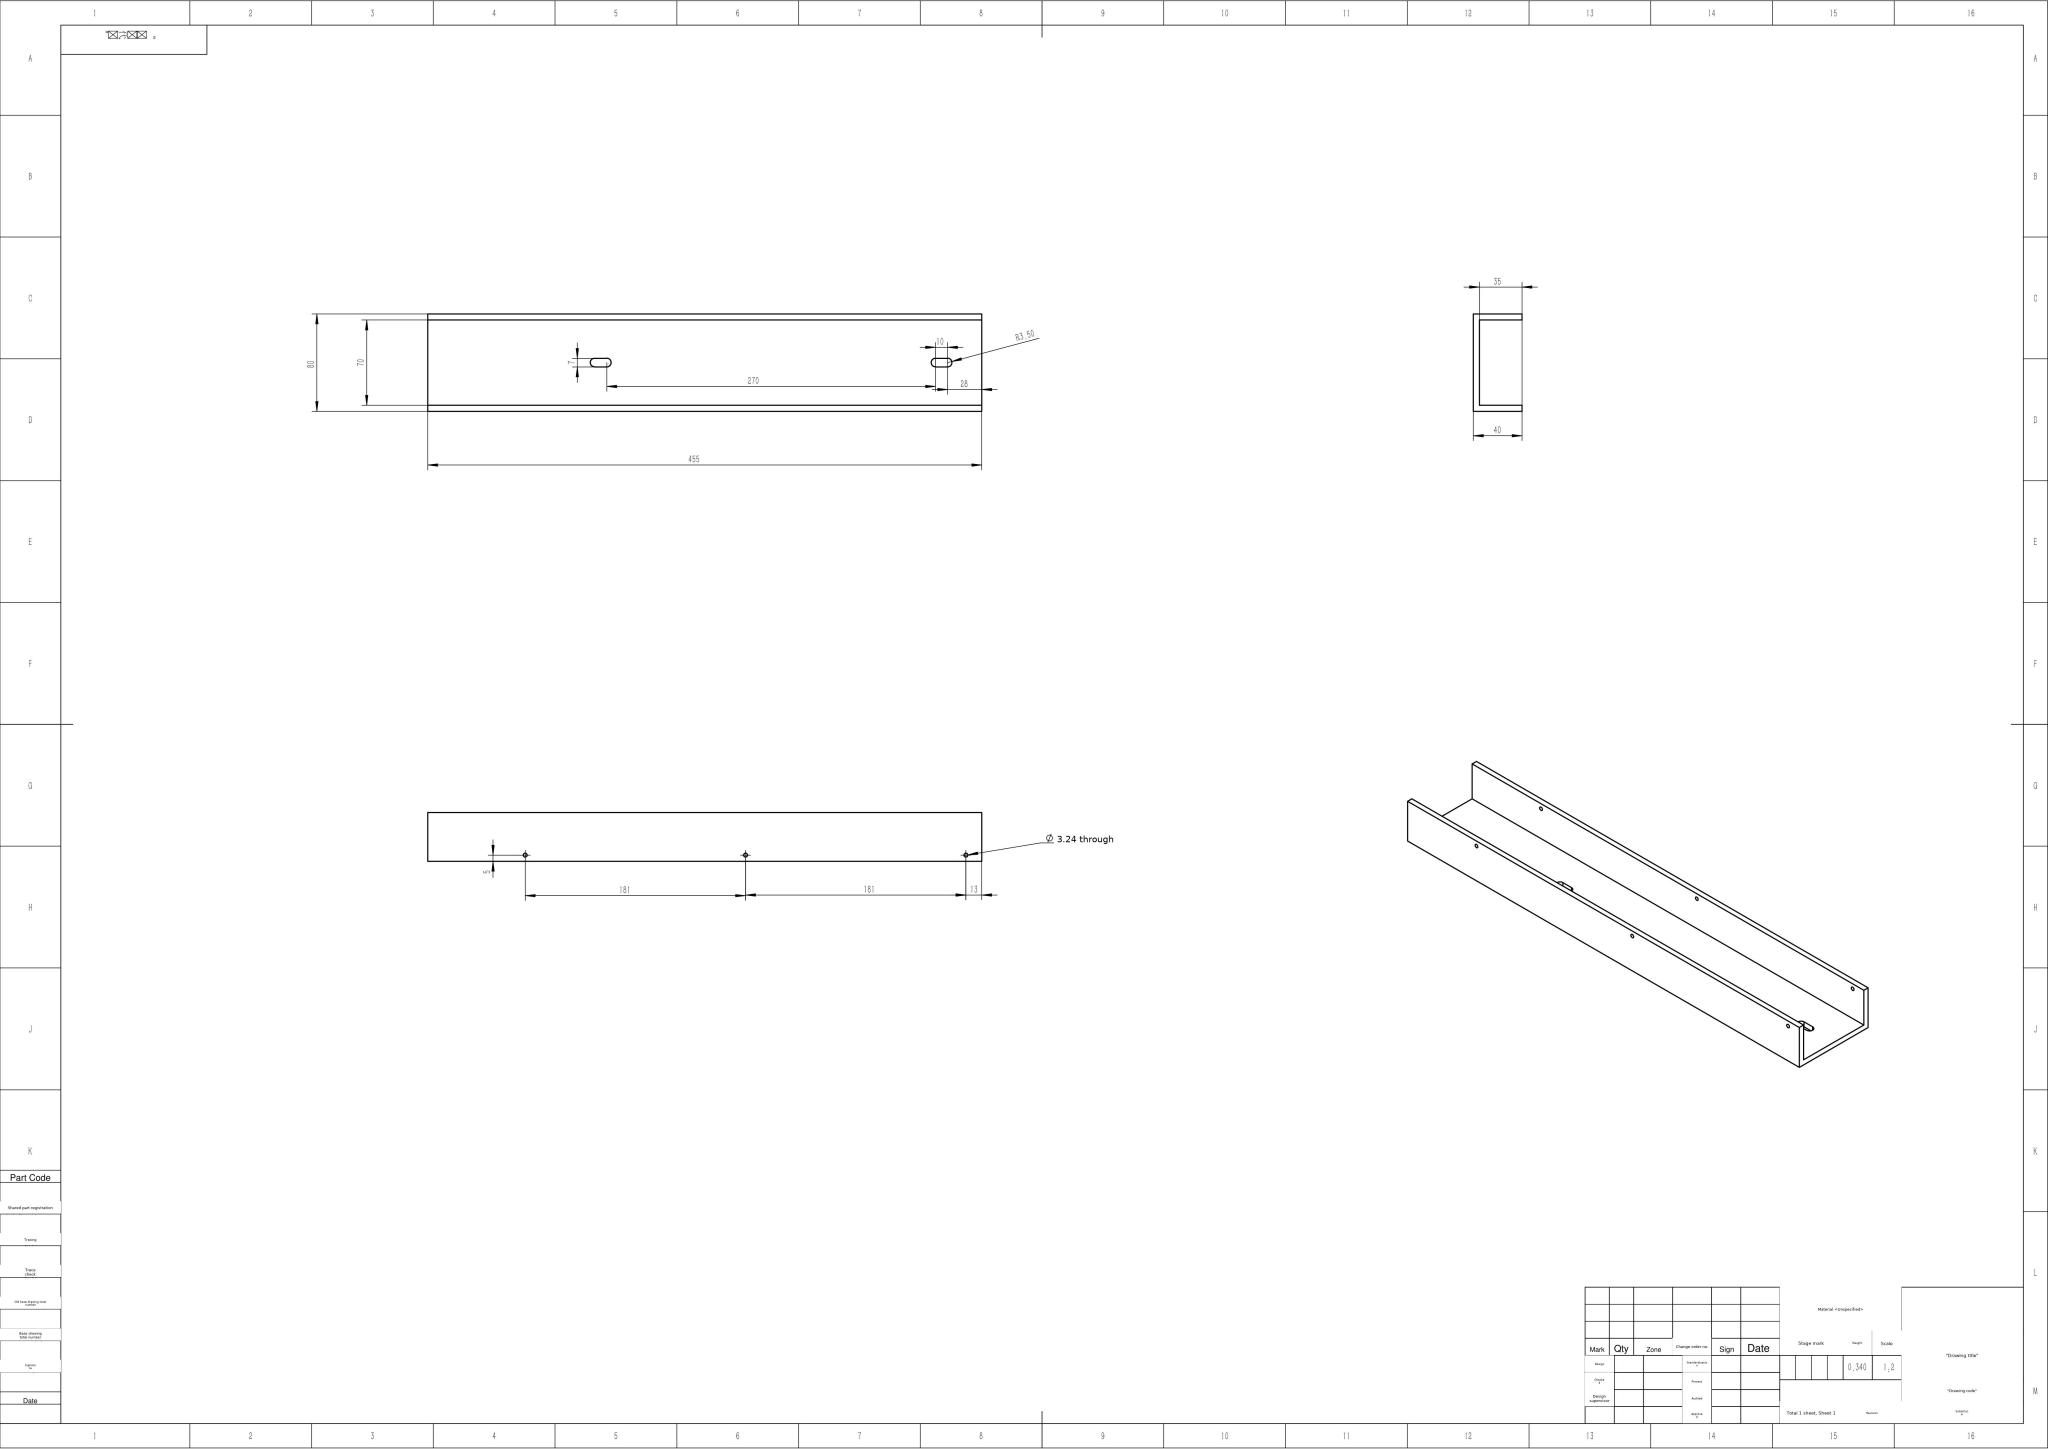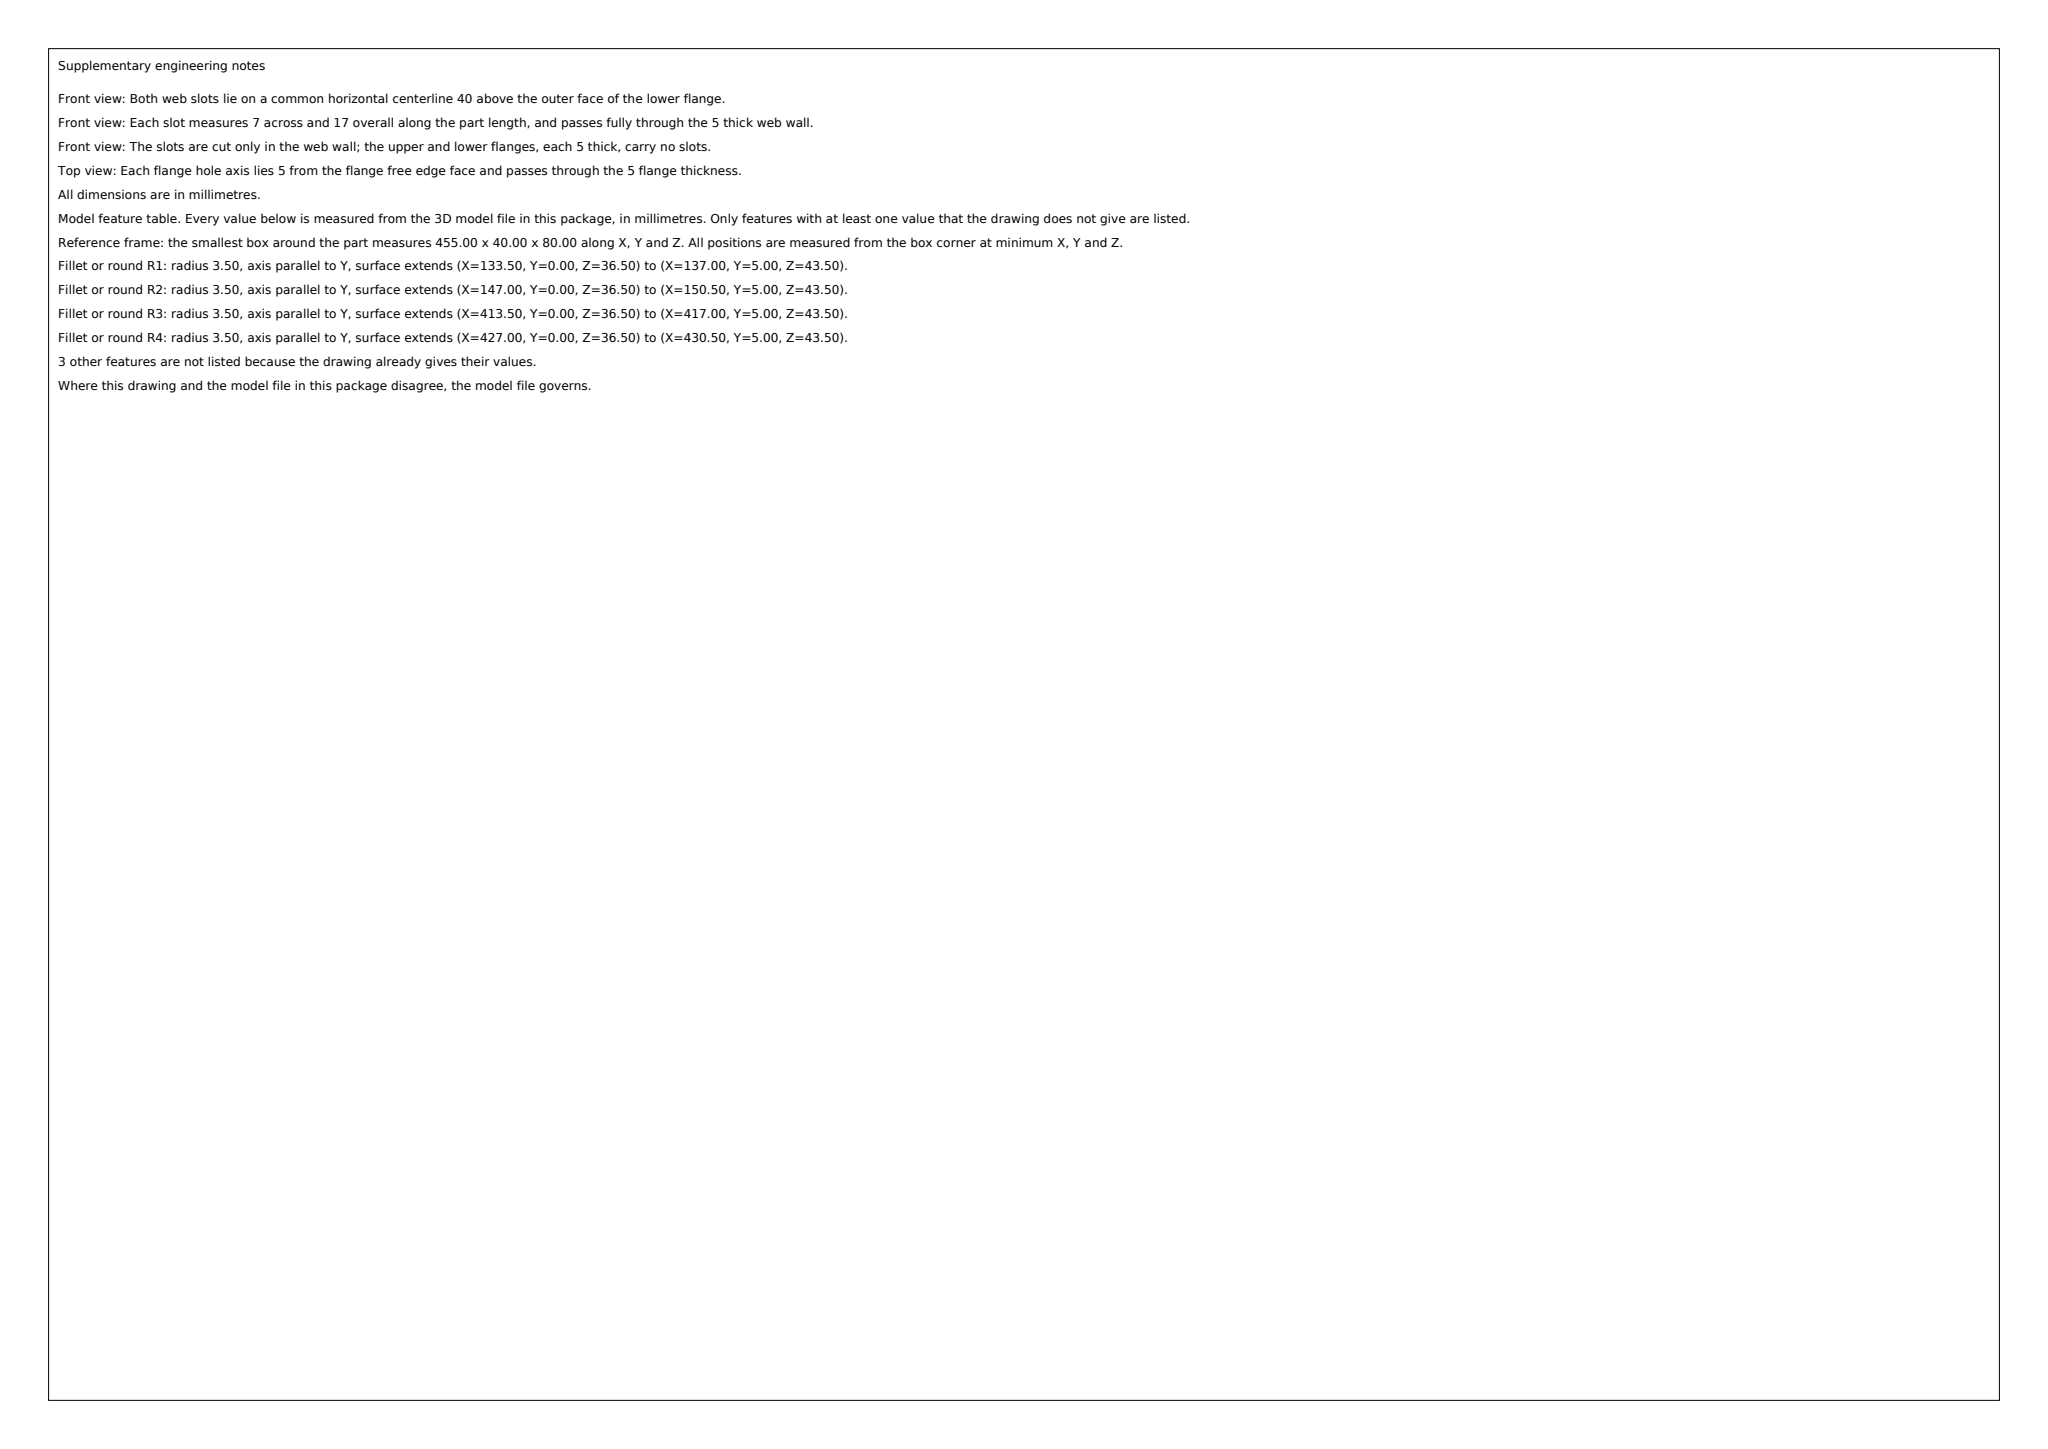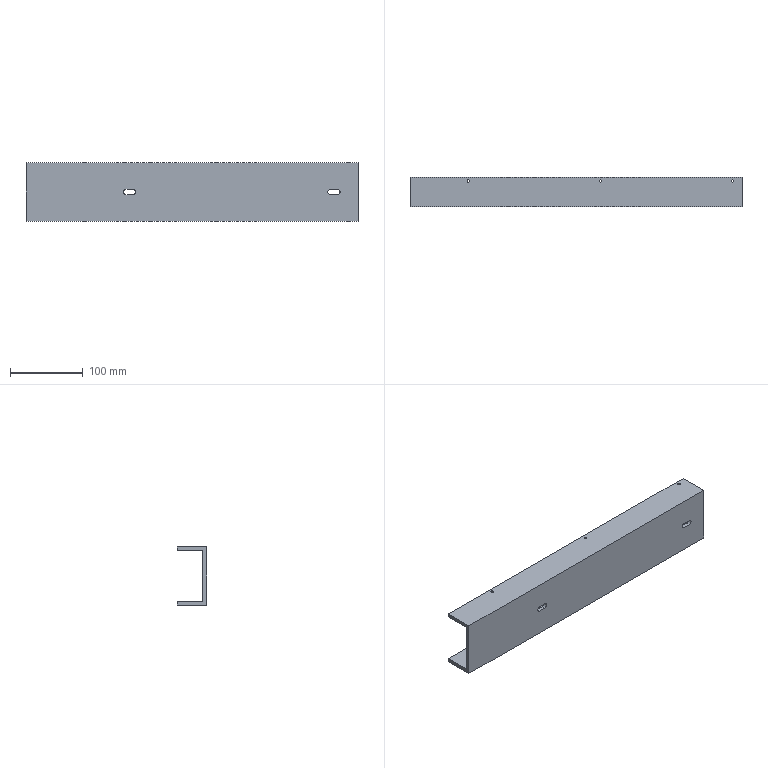Part | SolidWorks | mm | 1 solid | 30 faces | box 455 x 40 x 80 mm | volume 339917 mm3 | cylinder 16 | plane 14 | commonest cylinder face diameters 3.242 x12 7 x4
Drawing notes:
FLANGE THK 5 EA; 70 INNER SPAN 5 FROM EA OUTER FACE | from the solid: z-planes at 0, 5, 75, 80 over 80 overall height: 5 thk flange each end, 70 inner
2X 7 WIDE X 10 LG OBROUND SLOT THRU 5 WEB | from the solid: dia 7 cyls, axis y, length 5 (= web y 0-5), pairs at x=137/147 and x=417/427, z=40
2X OBROUND SLOT 7 WIDE X 10 LG: CL 40 FROM BOTTOM EDGE | from the solid: 7 dia y-axis cyls at z=40.0 (pos_other_axes [x,null,40.0]); bbox height 80.0 so CL is symmetric